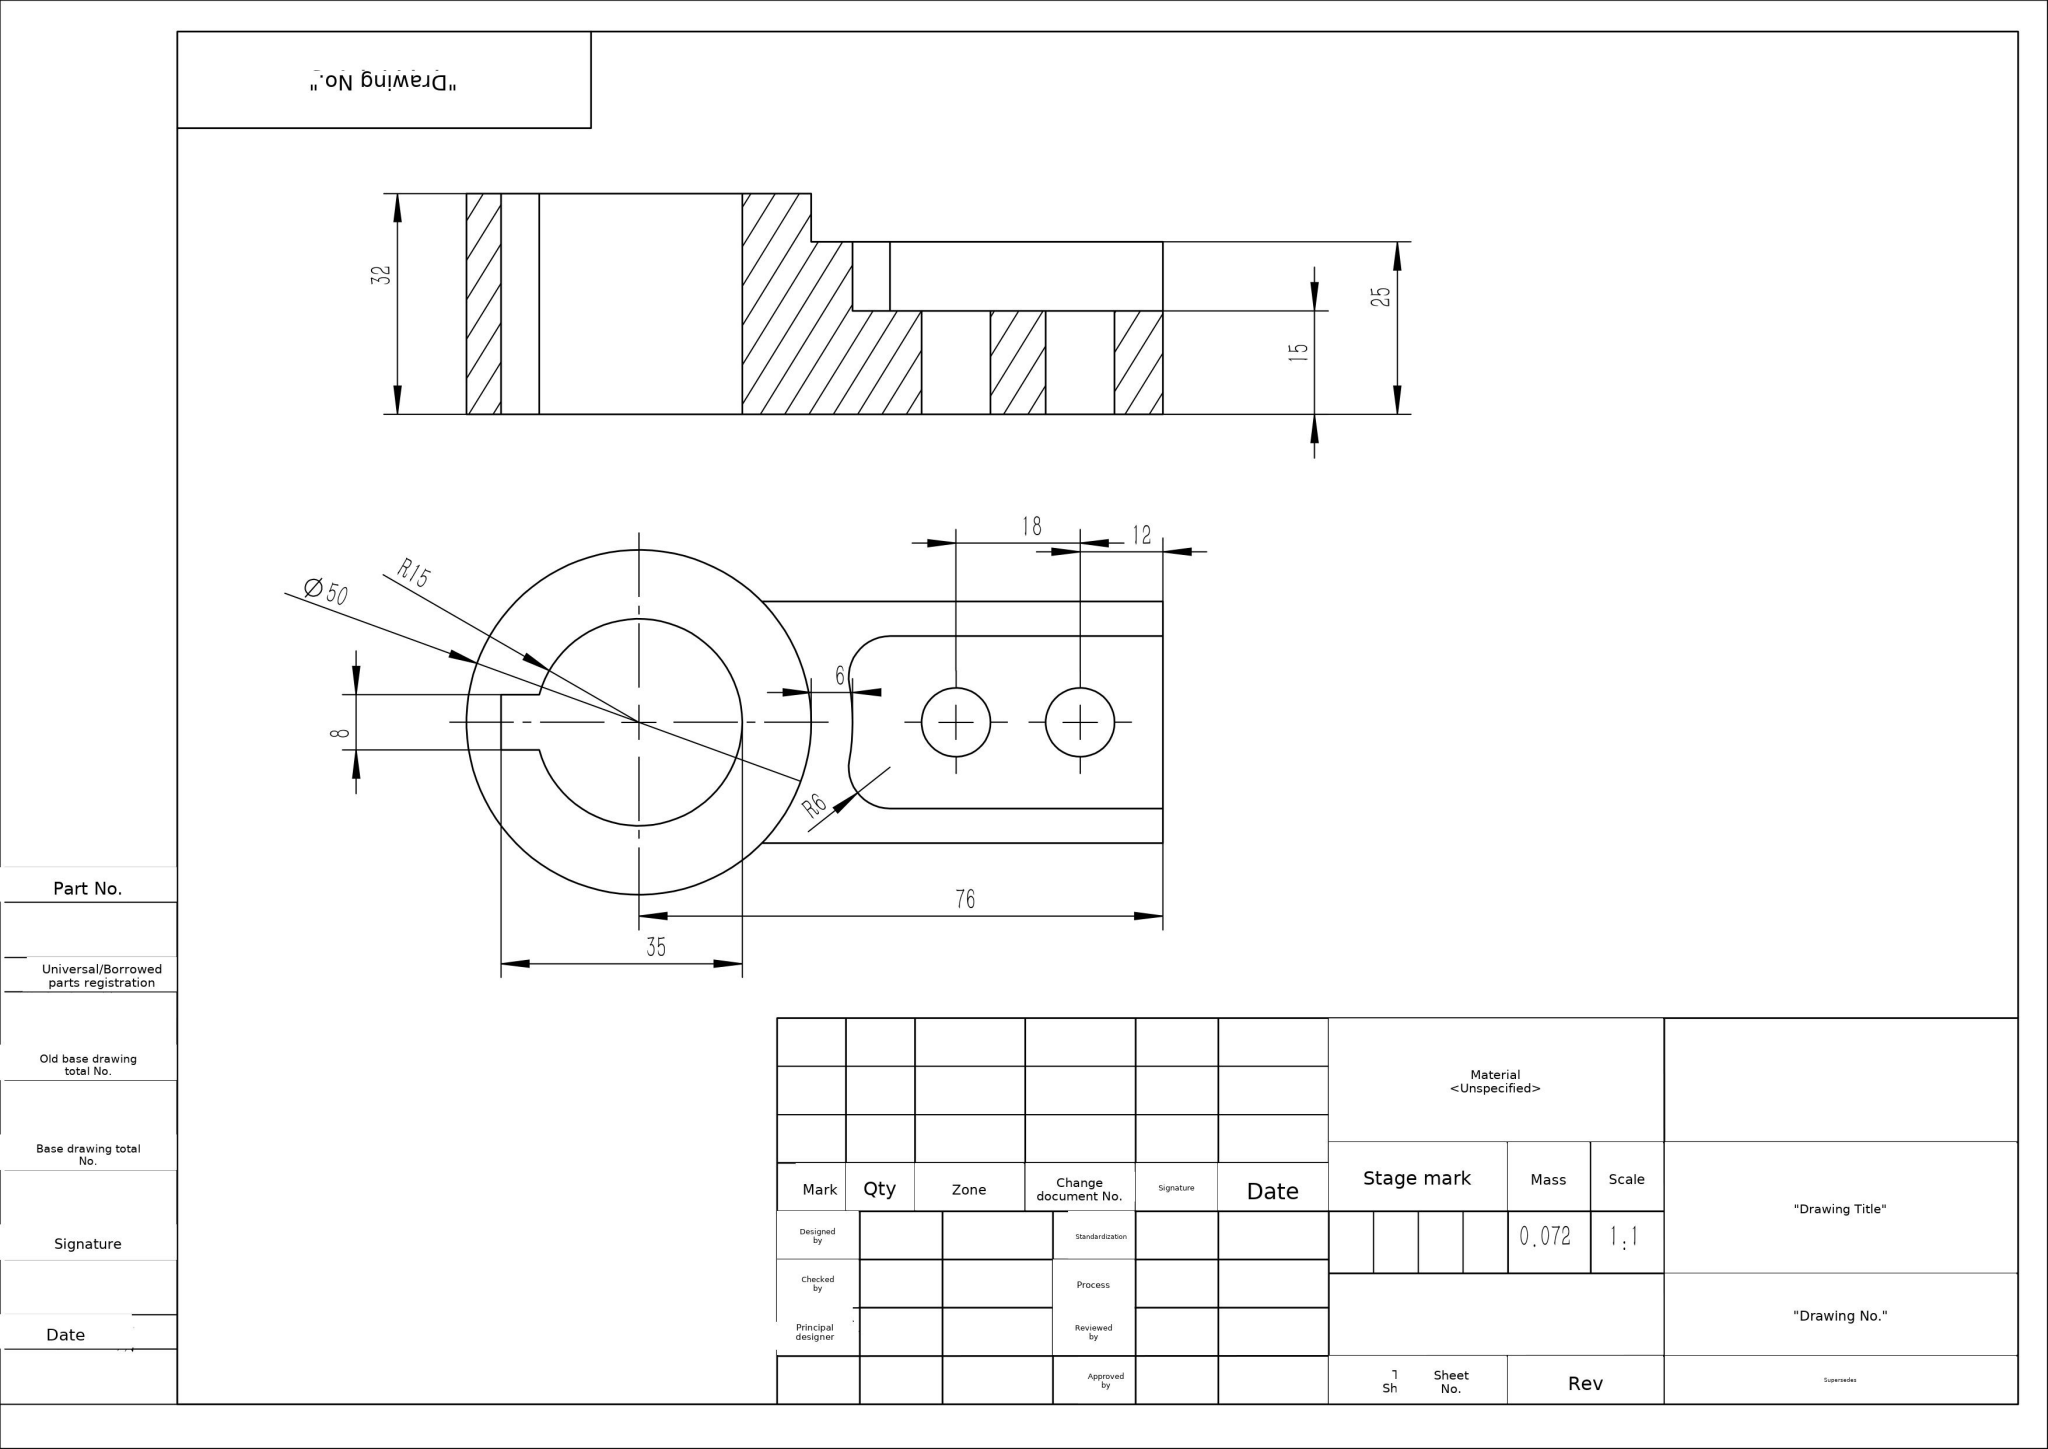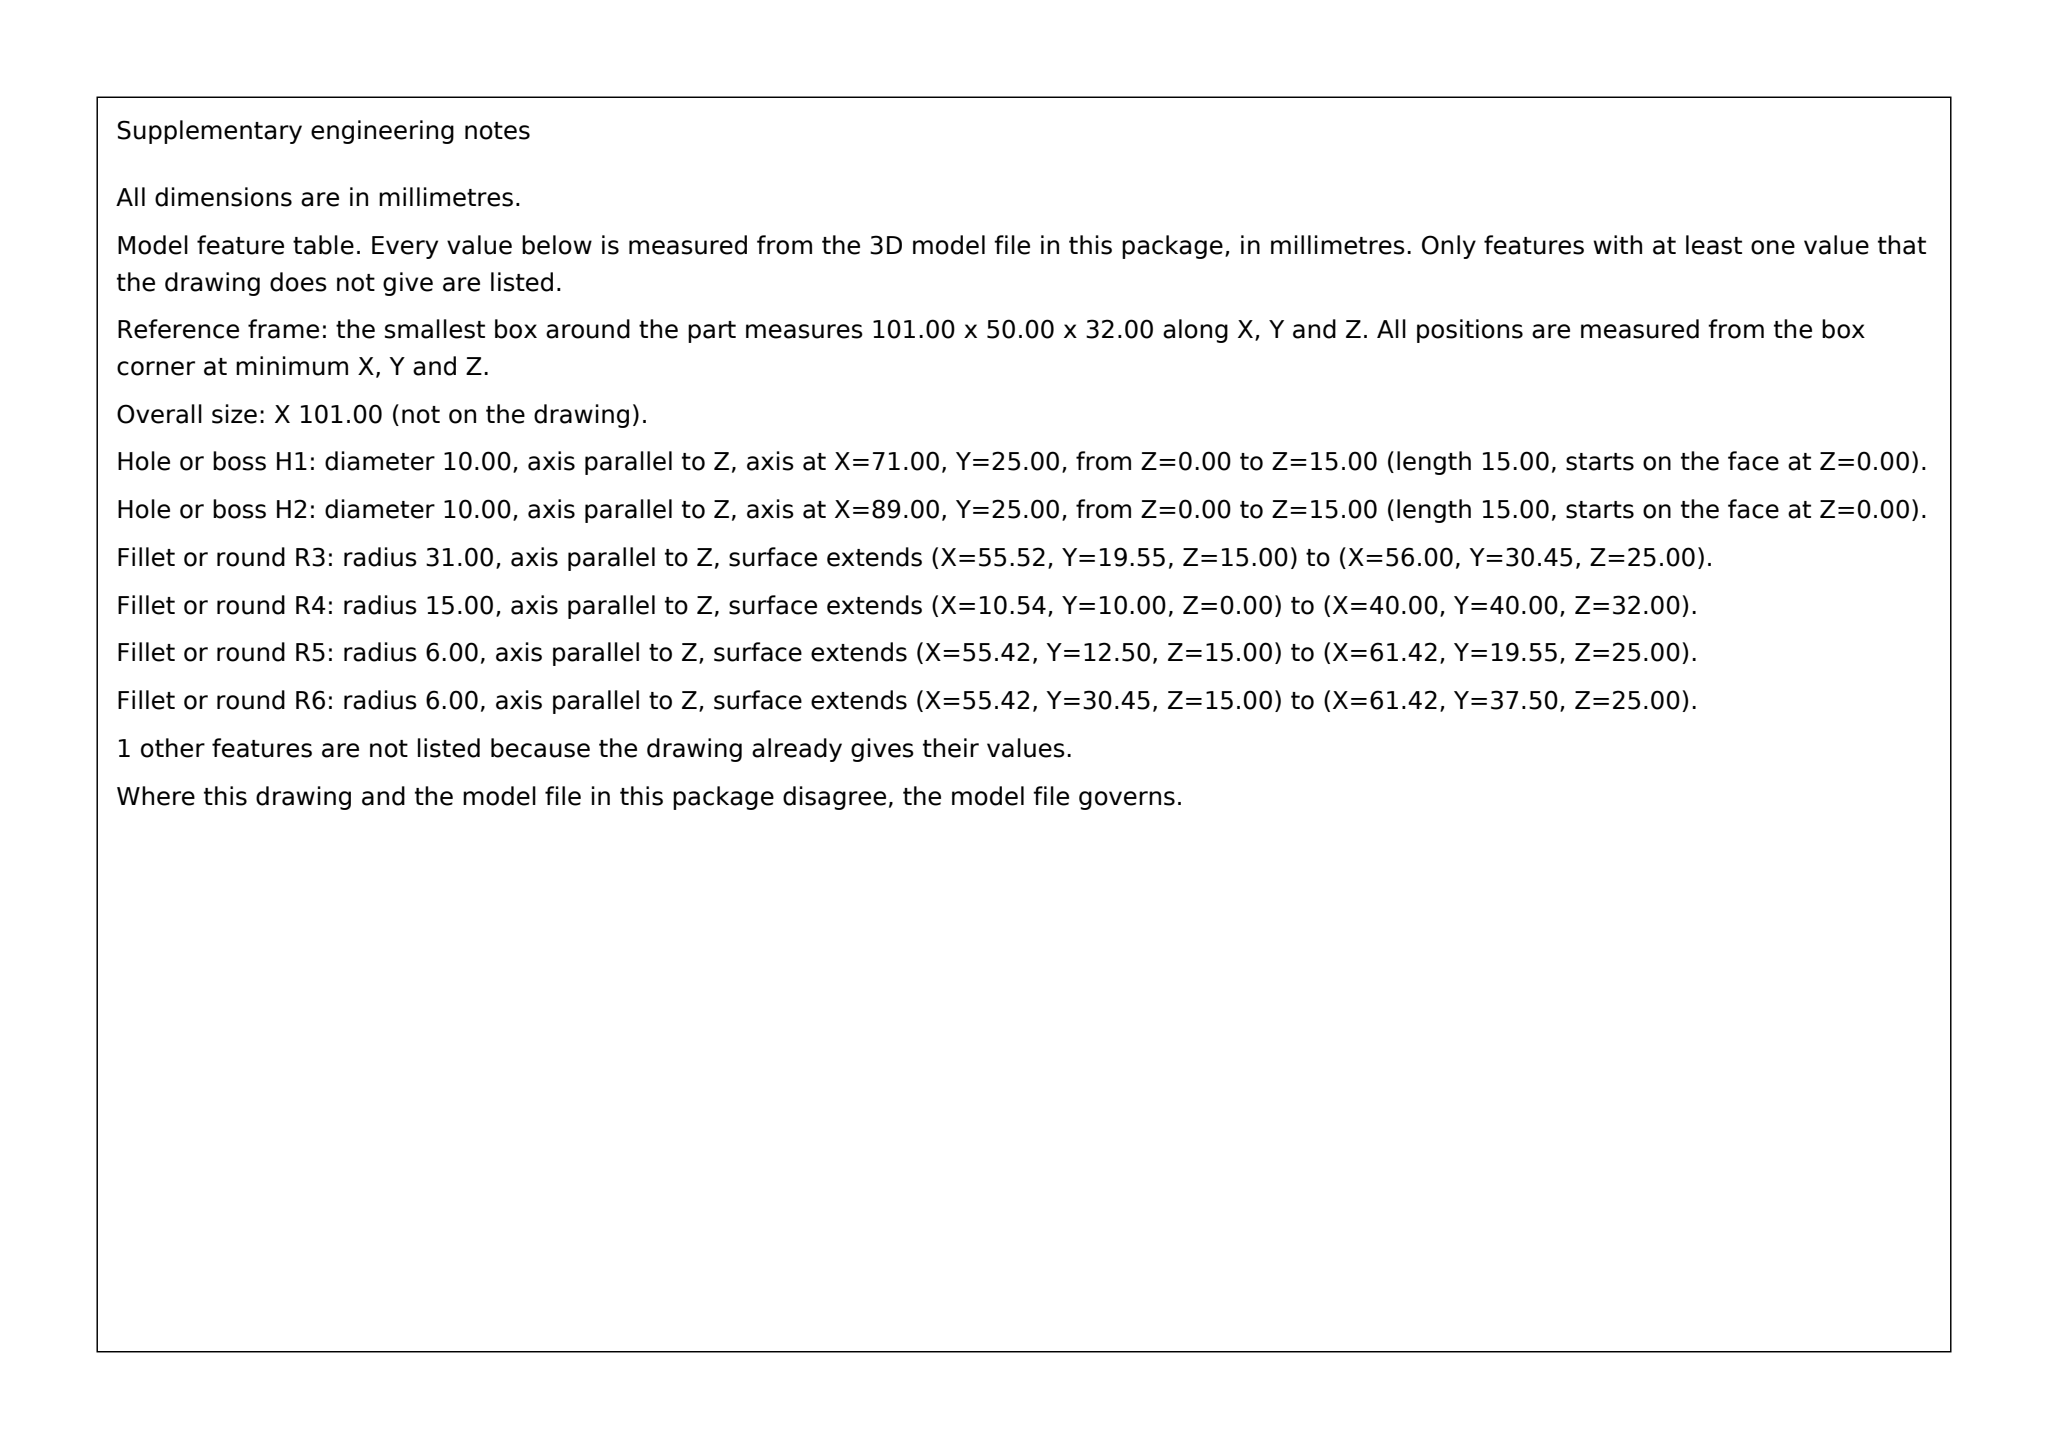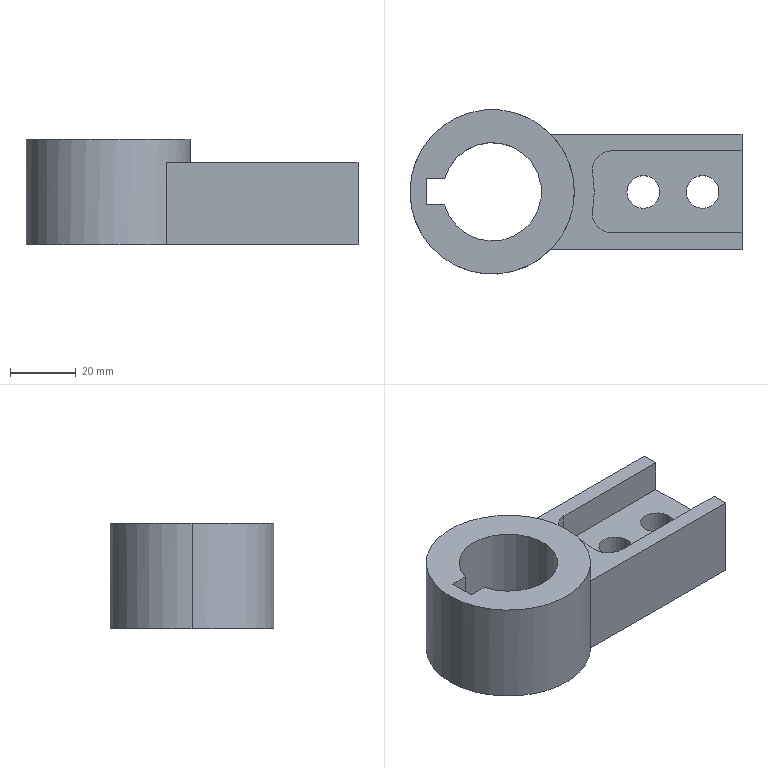Part | SolidWorks | mm | 1 solid | 23 faces | box 101 x 50 x 32 mm | volume 71910 mm3 | plane 12 | cylinder 11 | commonest cylinder face diameters 10 x4 62 x2 50 x2 12 x2 30 x1
build123d program:
from build123d import *

# Parameters (mm, degrees)
SKETCH1_R           = 25
BOSS_EXTRUDE1_DEPTH = 32
SKETCH2_W           = 61
SKETCH2_H           = 35
BOSS_EXTRUDE2_DEPTH = 25
CUT_EXTRUDE1_DEPTH  = 10
SKETCH4_R           = 5
CUT_EXTRUDE2_DEPTH  = 28


with BuildPart() as part:
    # Sketch1 → Boss-Extrude1 (new body)
    with BuildSketch(Plane.XY):
        Circle(SKETCH1_R)
        with BuildLine():
            Line((-14.457, 4), (-20, 4))
            Line((-20, 4), (-20, -4))
            Line((-20, -4), (-14.457, -4))
            ThreePointArc((-14.457, -4), (15, 0), (-14.457, 4))
        make_face(mode=Mode.SUBTRACT)
    extrude(amount=BOSS_EXTRUDE1_DEPTH)

    # Sketch2 → Boss-Extrude2 (add)
    with BuildSketch(Plane(origin=(0, 0, 0), x_dir=(-1, 0, 0), z_dir=(0, 0, -1))):
        with Locations((-45.5, 0)):
            Rectangle(SKETCH2_W, SKETCH2_H)
    extrude(amount=-BOSS_EXTRUDE2_DEPTH)

    # Sketch3 → Cut-Extrude1 (cut)
    with BuildSketch(Plane.XY.offset(25)):
        with BuildLine():
            Line((76, -12.5), (76, 12.5))
            Line((76, 12.5), (36.425, 12.5))
            ThreePointArc((36.425, 12.5), (31.824, 10.352), (30.518, 5.446))
            ThreePointArc((30.518, 5.446), (31, 0), (30.518, -5.446))
            ThreePointArc((30.518, -5.446), (31.824, -10.352), (36.425, -12.5))
            Line((36.425, -12.5), (76, -12.5))
        make_face()
    extrude(amount=-CUT_EXTRUDE1_DEPTH, mode=Mode.SUBTRACT)

    # Sketch4 → Cut-Extrude2 (cut)
    with BuildSketch(Plane.XY.offset(15)):
        with Locations((46, 0)):
            Circle(SKETCH4_R)
        with Locations((64, 0)):
            Circle(SKETCH4_R)
    extrude(amount=-CUT_EXTRUDE2_DEPTH, mode=Mode.SUBTRACT)


solid = part.part
STEP:
#1=CARTESIAN_POINT('',(59.,0.,0.));
#2=VERTEX_POINT('',#1);
#3=CARTESIAN_POINT('',(69.,0.,0.));
#4=VERTEX_POINT('',#3);
#5=CARTESIAN_POINT('',(64.,0.,0.));
#6=DIRECTION('',(0.,0.,1.));
#7=DIRECTION('',(1.,0.,0.));
#8=AXIS2_PLACEMENT_3D('',#5,#6,#7);
#9=CIRCLE('',#8,5.);
#10=EDGE_CURVE('',#2,#4,#9,.T.);
#11=ORIENTED_EDGE('',*,*,#10,.F.);
#12=CARTESIAN_POINT('',(59.,0.,15.));
#13=VERTEX_POINT('',#12);
#14=CARTESIAN_POINT('',(59.,0.,-13.));
#15=DIRECTION('',(0.,0.,1.));
#16=VECTOR('',#15,1000.);
#17=LINE('',#14,#16);
#18=EDGE_CURVE('',#2,#13,#17,.T.);
#19=ORIENTED_EDGE('',*,*,#18,.T.);
#20=CARTESIAN_POINT('',(69.,0.,15.));
#21=VERTEX_POINT('',#20);
#22=CARTESIAN_POINT('',(64.,0.,15.));
#23=DIRECTION('',(0.,0.,1.));
#24=DIRECTION('',(1.,0.,0.));
#25=AXIS2_PLACEMENT_3D('',#22,#23,#24);
#26=CIRCLE('',#25,5.);
#27=EDGE_CURVE('',#13,#21,#26,.T.);
#28=ORIENTED_EDGE('',*,*,#27,.T.);
#29=CARTESIAN_POINT('',(69.,0.,-13.));
#30=DIRECTION('',(0.,0.,1.));
#31=VECTOR('',#30,1000.);
#32=LINE('',#29,#31);
#33=EDGE_CURVE('',#4,#21,#32,.T.);
#34=ORIENTED_EDGE('',*,*,#33,.F.);
#35=EDGE_LOOP('',(#11,#19,#28,#34));
#36=FACE_OUTER_BOUND('',#35,.T.);
#37=CARTESIAN_POINT('',(64.,0.,-13.));
#38=DIRECTION('',(0.,0.,1.));
#39=DIRECTION('',(1.,0.,0.));
#40=AXIS2_PLACEMENT_3D('',#37,#38,#39);
#41=CYLINDRICAL_SURFACE('',#40,5.);
#42=ADVANCED_FACE('',(#36),#41,.F.);
#43=CARTESIAN_POINT('',(41.,0.,0.));
#44=VERTEX_POINT('',#43);
#45=CARTESIAN_POINT('',(51.,0.,0.));
#46=VERTEX_POINT('',#45);
#47=CARTESIAN_POINT('',(46.,0.,0.));
#48=DIRECTION('',(0.,0.,1.));
#49=DIRECTION('',(1.,0.,0.));
#50=AXIS2_PLACEMENT_3D('',#47,#48,#49);
#51=CIRCLE('',#50,5.);
#52=EDGE_CURVE('',#44,#46,#51,.T.);
#53=ORIENTED_EDGE('',*,*,#52,.F.);
#54=CARTESIAN_POINT('',(41.,0.,15.));
#55=VERTEX_POINT('',#54);
#56=CARTESIAN_POINT('',(41.,0.,-13.));
#57=DIRECTION('',(0.,0.,1.));
#58=VECTOR('',#57,1000.);
#59=LINE('',#56,#58);
#60=EDGE_CURVE('',#44,#55,#59,.T.);
#61=ORIENTED_EDGE('',*,*,#60,.T.);
#62=CARTESIAN_POINT('',(51.,0.,15.));
#63=VERTEX_POINT('',#62);
#64=CARTESIAN_POINT('',(46.,0.,15.));
#65=DIRECTION('',(0.,0.,1.));
#66=DIRECTION('',(1.,0.,0.));
#67=AXIS2_PLACEMENT_3D('',#64,#65,#66);
#68=CIRCLE('',#67,5.);
#69=EDGE_CURVE('',#55,#63,#68,.T.);
#70=ORIENTED_EDGE('',*,*,#69,.T.);
#71=CARTESIAN_POINT('',(51.,0.,-13.));
#72=DIRECTION('',(0.,0.,1.));
#73=VECTOR('',#72,1000.);
#74=LINE('',#71,#73);
#75=EDGE_CURVE('',#46,#63,#74,.T.);
#76=ORIENTED_EDGE('',*,*,#75,.F.);
#77=EDGE_LOOP('',(#53,#61,#70,#76));
#78=FACE_OUTER_BOUND('',#77,.T.);
#79=CARTESIAN_POINT('',(46.,0.,-13.));
#80=DIRECTION('',(0.,0.,1.));
#81=DIRECTION('',(1.,0.,0.));
#82=AXIS2_PLACEMENT_3D('',#79,#80,#81);
#83=CYLINDRICAL_SURFACE('',#82,5.);
#84=ADVANCED_FACE('',(#78),#83,.F.);
#85=CARTESIAN_POINT('',(30.518,-5.446,15.));
#86=VERTEX_POINT('',#85);
#87=CARTESIAN_POINT('',(31.,0.,15.));
#88=VERTEX_POINT('',#87);
#89=CARTESIAN_POINT('',(0.,0.,15.));
#90=DIRECTION('',(0.,0.,1.));
#91=DIRECTION('',(1.,0.,0.));
#92=AXIS2_PLACEMENT_3D('',#89,#90,#91);
#93=CIRCLE('',#92,31.);
#94=EDGE_CURVE('',#86,#88,#93,.T.);
#95=ORIENTED_EDGE('',*,*,#94,.T.);
#96=CARTESIAN_POINT('',(31.,0.,25.));
#97=VERTEX_POINT('',#96);
#98=CARTESIAN_POINT('',(31.,0.,15.));
#99=DIRECTION('',(0.,0.,1.));
#100=VECTOR('',#99,1000.);
#101=LINE('',#98,#100);
#102=EDGE_CURVE('',#88,#97,#101,.T.);
#103=ORIENTED_EDGE('',*,*,#102,.T.);
#104=CARTESIAN_POINT('',(30.518,-5.446,25.));
#105=VERTEX_POINT('',#104);
#106=CARTESIAN_POINT('',(0.,0.,25.));
#107=DIRECTION('',(0.,0.,1.));
#108=DIRECTION('',(1.,0.,0.));
#109=AXIS2_PLACEMENT_3D('',#106,#107,#108);
#110=CIRCLE('',#109,31.);
#111=EDGE_CURVE('',#105,#97,#110,.T.);
#112=ORIENTED_EDGE('',*,*,#111,.F.);
#113=CARTESIAN_POINT('',(30.518,-5.446,15.));
#114=DIRECTION('',(0.,0.,1.));
#115=VECTOR('',#114,1000.);
#116=LINE('',#113,#115);
#117=EDGE_CURVE('',#86,#105,#116,.T.);
#118=ORIENTED_EDGE('',*,*,#117,.F.);
#119=EDGE_LOOP('',(#95,#103,#112,#118));
#120=FACE_OUTER_BOUND('',#119,.T.);
#121=CARTESIAN_POINT('',(0.,0.,15.));
#122=DIRECTION('',(0.,0.,1.));
#123=DIRECTION('',(1.,0.,0.));
#124=AXIS2_PLACEMENT_3D('',#121,#122,#123);
#125=CYLINDRICAL_SURFACE('',#124,31.);
#126=ADVANCED_FACE('',(#120),#125,.T.);
#127=CARTESIAN_POINT('',(25.,0.,32.));
#128=VERTEX_POINT('',#127);
#129=CARTESIAN_POINT('',(-25.,0.,32.));
#130=VERTEX_POINT('',#129);
#131=CARTESIAN_POINT('',(0.,0.,32.));
#132=DIRECTION('',(0.,0.,1.));
#133=DIRECTION('',(1.,0.,0.));
#134=AXIS2_PLACEMENT_3D('',#131,#132,#133);
#135=CIRCLE('',#134,25.);
#136=EDGE_CURVE('',#128,#130,#135,.T.);
#137=ORIENTED_EDGE('',*,*,#136,.F.);
#138=CARTESIAN_POINT('',(25.,0.,25.));
#139=VERTEX_POINT('',#138);
#140=CARTESIAN_POINT('',(25.,0.,32.));
#141=DIRECTION('',(0.,0.,-1.));
#142=VECTOR('',#141,1000.);
#143=LINE('',#140,#142);
#144=EDGE_CURVE('',#128,#139,#143,.T.);
#145=ORIENTED_EDGE('',*,*,#144,.T.);
#146=CARTESIAN_POINT('',(17.854,17.5,25.));
#147=VERTEX_POINT('',#146);
#148=CARTESIAN_POINT('',(0.,0.,25.));
#149=DIRECTION('',(0.,0.,1.));
#150=DIRECTION('',(1.,0.,0.));
#151=AXIS2_PLACEMENT_3D('',#148,#149,#150);
#152=CIRCLE('',#151,25.);
#153=EDGE_CURVE('',#139,#147,#152,.T.);
#154=ORIENTED_EDGE('',*,*,#153,.T.);
#155=CARTESIAN_POINT('',(17.854,17.5,0.));
#156=VERTEX_POINT('',#155);
#157=CARTESIAN_POINT('',(17.854,17.5,32.));
#158=DIRECTION('',(0.,0.,-1.));
#159=VECTOR('',#158,1000.);
#160=LINE('',#157,#159);
#161=EDGE_CURVE('',#147,#156,#160,.T.);
#162=ORIENTED_EDGE('',*,*,#161,.T.);
#163=CARTESIAN_POINT('',(-25.,0.,0.));
#164=VERTEX_POINT('',#163);
#165=CARTESIAN_POINT('',(0.,0.,0.));
#166=DIRECTION('',(0.,0.,1.));
#167=DIRECTION('',(1.,0.,0.));
#168=AXIS2_PLACEMENT_3D('',#165,#166,#167);
#169=CIRCLE('',#168,25.);
#170=EDGE_CURVE('',#156,#164,#169,.T.);
#171=ORIENTED_EDGE('',*,*,#170,.T.);
#172=CARTESIAN_POINT('',(-25.,0.,32.));
#173=DIRECTION('',(0.,0.,-1.));
#174=VECTOR('',#173,1000.);
#175=LINE('',#172,#174);
#176=EDGE_CURVE('',#130,#164,#175,.T.);
#177=ORIENTED_EDGE('',*,*,#176,.F.);
#178=EDGE_LOOP('',(#137,#145,#154,#162,#171,#177));
#179=FACE_OUTER_BOUND('',#178,.T.);
#180=CARTESIAN_POINT('',(0.,0.,32.));
#181=DIRECTION('',(0.,0.,-1.));
#182=DIRECTION('',(-1.,0.,0.));
#183=AXIS2_PLACEMENT_3D('',#180,#181,#182);
#184=CYLINDRICAL_SURFACE('',#183,25.);
#185=ADVANCED_FACE('',(#179),#184,.T.);
#186=CARTESIAN_POINT('',(0.,0.,32.));
#187=DIRECTION('',(0.,0.,1.));
#188=DIRECTION('',(1.,0.,0.));
#189=AXIS2_PLACEMENT_3D('',#186,#187,#188);
#190=CIRCLE('',#189,25.);
#191=EDGE_CURVE('',#130,#128,#190,.T.);
#192=ORIENTED_EDGE('',*,*,#191,.T.);
#193=ORIENTED_EDGE('',*,*,#136,.T.);
#194=EDGE_LOOP('',(#192,#193));
#195=FACE_OUTER_BOUND('',#194,.T.);
#196=CARTESIAN_POINT('',(-20.,-4.,32.));
#197=VERTEX_POINT('',#196);
#198=CARTESIAN_POINT('',(-14.457,-4.,32.));
#199=VERTEX_POINT('',#198);
#200=CARTESIAN_POINT('',(-14.457,-4.,32.));
#201=DIRECTION('',(1.,0.,0.));
#202=VECTOR('',#201,1000.);
#203=LINE('',#200,#202);
#204=EDGE_CURVE('',#197,#199,#203,.T.);
#205=ORIENTED_EDGE('',*,*,#204,.F.);
#206=CARTESIAN_POINT('',(-20.,4.,32.));
#207=VERTEX_POINT('',#206);
#208=CARTESIAN_POINT('',(-20.,4.,32.));
#209=DIRECTION('',(0.,-1.,0.));
#210=VECTOR('',#209,1000.);
#211=LINE('',#208,#210);
#212=EDGE_CURVE('',#207,#197,#211,.T.);
#213=ORIENTED_EDGE('',*,*,#212,.F.);
#214=CARTESIAN_POINT('',(-14.457,4.,32.));
#215=VERTEX_POINT('',#214);
#216=CARTESIAN_POINT('',(-14.457,4.,32.));
#217=DIRECTION('',(-1.,-0.,0.));
#218=VECTOR('',#217,1000.);
#219=LINE('',#216,#218);
#220=EDGE_CURVE('',#215,#207,#219,.T.);
#221=ORIENTED_EDGE('',*,*,#220,.F.);
#222=CARTESIAN_POINT('',(0.,0.,32.));
#223=DIRECTION('',(0.,0.,1.));
#224=DIRECTION('',(1.,0.,0.));
#225=AXIS2_PLACEMENT_3D('',#222,#223,#224);
#226=CIRCLE('',#225,15.);
#227=EDGE_CURVE('',#199,#215,#226,.T.);
#228=ORIENTED_EDGE('',*,*,#227,.F.);
#229=EDGE_LOOP('',(#205,#213,#221,#228));
#230=FACE_BOUND('',#229,.T.);
#231=CARTESIAN_POINT('',(0.,0.,32.));
#232=DIRECTION('',(0.,0.,1.));
#233=DIRECTION('',(1.,0.,0.));
#234=AXIS2_PLACEMENT_3D('',#231,#232,#233);
#235=PLANE('',#234);
#236=ADVANCED_FACE('',(#195,#230),#235,.T.);
#237=CARTESIAN_POINT('',(64.,0.,0.));
#238=DIRECTION('',(0.,0.,1.));
#239=DIRECTION('',(1.,0.,0.));
#240=AXIS2_PLACEMENT_3D('',#237,#238,#239);
#241=CIRCLE('',#240,5.);
#242=EDGE_CURVE('',#4,#2,#241,.T.);
#243=ORIENTED_EDGE('',*,*,#242,.T.);
#244=ORIENTED_EDGE('',*,*,#10,.T.);
#245=EDGE_LOOP('',(#243,#244));
#246=FACE_BOUND('',#245,.T.);
#247=CARTESIAN_POINT('',(46.,0.,0.));
#248=DIRECTION('',(0.,0.,1.));
#249=DIRECTION('',(1.,0.,0.));
#250=AXIS2_PLACEMENT_3D('',#247,#248,#249);
#251=CIRCLE('',#250,5.);
#252=EDGE_CURVE('',#46,#44,#251,.T.);
#253=ORIENTED_EDGE('',*,*,#252,.T.);
#254=ORIENTED_EDGE('',*,*,#52,.T.);
#255=EDGE_LOOP('',(#253,#254));
#256=FACE_BOUND('',#255,.T.);
#257=CARTESIAN_POINT('',(-14.457,-4.,0.));
#258=VERTEX_POINT('',#257);
#259=CARTESIAN_POINT('',(-14.457,4.,0.));
#260=VERTEX_POINT('',#259);
#261=CARTESIAN_POINT('',(0.,0.,0.));
#262=DIRECTION('',(0.,0.,1.));
#263=DIRECTION('',(1.,0.,0.));
#264=AXIS2_PLACEMENT_3D('',#261,#262,#263);
#265=CIRCLE('',#264,15.);
#266=EDGE_CURVE('',#258,#260,#265,.T.);
#267=ORIENTED_EDGE('',*,*,#266,.T.);
#268=CARTESIAN_POINT('',(-20.,4.,0.));
#269=VERTEX_POINT('',#268);
#270=CARTESIAN_POINT('',(-14.457,4.,0.));
#271=DIRECTION('',(-1.,-0.,0.));
#272=VECTOR('',#271,1000.);
#273=LINE('',#270,#272);
#274=EDGE_CURVE('',#260,#269,#273,.T.);
#275=ORIENTED_EDGE('',*,*,#274,.T.);
#276=CARTESIAN_POINT('',(-20.,-4.,0.));
#277=VERTEX_POINT('',#276);
#278=CARTESIAN_POINT('',(-20.,4.,0.));
#279=DIRECTION('',(0.,-1.,0.));
#280=VECTOR('',#279,1000.);
#281=LINE('',#278,#280);
#282=EDGE_CURVE('',#269,#277,#281,.T.);
#283=ORIENTED_EDGE('',*,*,#282,.T.);
#284=CARTESIAN_POINT('',(-14.457,-4.,0.));
#285=DIRECTION('',(1.,0.,0.));
#286=VECTOR('',#285,1000.);
#287=LINE('',#284,#286);
#288=EDGE_CURVE('',#277,#258,#287,.T.);
#289=ORIENTED_EDGE('',*,*,#288,.T.);
#290=EDGE_LOOP('',(#267,#275,#283,#289));
#291=FACE_BOUND('',#290,.T.);
#292=CARTESIAN_POINT('',(76.,-17.5,0.));
#293=VERTEX_POINT('',#292);
#294=CARTESIAN_POINT('',(17.854,-17.5,0.));
#295=VERTEX_POINT('',#294);
#296=CARTESIAN_POINT('',(15.,-17.5,0.));
#297=DIRECTION('',(-1.,0.,0.));
#298=VECTOR('',#297,1000.);
#299=LINE('',#296,#298);
#300=EDGE_CURVE('',#293,#295,#299,.T.);
#301=ORIENTED_EDGE('',*,*,#300,.T.);
#302=CARTESIAN_POINT('',(0.,0.,0.));
#303=DIRECTION('',(0.,0.,1.));
#304=DIRECTION('',(1.,0.,0.));
#305=AXIS2_PLACEMENT_3D('',#302,#303,#304);
#306=CIRCLE('',#305,25.);
#307=EDGE_CURVE('',#164,#295,#306,.T.);
#308=ORIENTED_EDGE('',*,*,#307,.F.);
#309=ORIENTED_EDGE('',*,*,#170,.F.);
#310=CARTESIAN_POINT('',(76.,17.5,0.));
#311=VERTEX_POINT('',#310);
#312=CARTESIAN_POINT('',(15.,17.5,0.));
#313=DIRECTION('',(1.,0.,0.));
#314=VECTOR('',#313,1000.);
#315=LINE('',#312,#314);
#316=EDGE_CURVE('',#156,#311,#315,.T.);
#317=ORIENTED_EDGE('',*,*,#316,.T.);
#318=CARTESIAN_POINT('',(76.,17.5,0.));
#319=DIRECTION('',(0.,-1.,0.));
#320=VECTOR('',#319,1000.);
#321=LINE('',#318,#320);
#322=EDGE_CURVE('',#311,#293,#321,.T.);
#323=ORIENTED_EDGE('',*,*,#322,.T.);
#324=EDGE_LOOP('',(#301,#308,#309,#317,#323));
#325=FACE_OUTER_BOUND('',#324,.T.);
#326=CARTESIAN_POINT('',(0.,0.,0.));
#327=DIRECTION('',(0.,0.,1.));
#328=DIRECTION('',(1.,0.,0.));
#329=AXIS2_PLACEMENT_3D('',#326,#327,#328);
#330=PLANE('',#329);
#331=ADVANCED_FACE('',(#246,#256,#291,#325),#330,.F.);
#332=ORIENTED_EDGE('',*,*,#144,.F.);
#333=ORIENTED_EDGE('',*,*,#191,.F.);
#334=ORIENTED_EDGE('',*,*,#176,.T.);
#335=ORIENTED_EDGE('',*,*,#307,.T.);
#336=CARTESIAN_POINT('',(17.854,-17.5,25.));
#337=VERTEX_POINT('',#336);
#338=CARTESIAN_POINT('',(17.854,-17.5,32.));
#339=DIRECTION('',(0.,0.,1.));
#340=VECTOR('',#339,1000.);
#341=LINE('',#338,#340);
#342=EDGE_CURVE('',#295,#337,#341,.T.);
#343=ORIENTED_EDGE('',*,*,#342,.T.);
#344=CARTESIAN_POINT('',(0.,0.,25.));
#345=DIRECTION('',(0.,0.,1.));
#346=DIRECTION('',(1.,0.,0.));
#347=AXIS2_PLACEMENT_3D('',#344,#345,#346);
#348=CIRCLE('',#347,25.);
#349=EDGE_CURVE('',#337,#139,#348,.T.);
#350=ORIENTED_EDGE('',*,*,#349,.T.);
#351=EDGE_LOOP('',(#332,#333,#334,#335,#343,#350));
#352=FACE_OUTER_BOUND('',#351,.T.);
#353=CARTESIAN_POINT('',(0.,0.,32.));
#354=DIRECTION('',(0.,0.,-1.));
#355=DIRECTION('',(-1.,0.,0.));
#356=AXIS2_PLACEMENT_3D('',#353,#354,#355);
#357=CYLINDRICAL_SURFACE('',#356,25.);
#358=ADVANCED_FACE('',(#352),#357,.T.);
#359=ORIENTED_EDGE('',*,*,#282,.F.);
#360=CARTESIAN_POINT('',(-20.,4.,32.));
#361=DIRECTION('',(0.,0.,-1.));
#362=VECTOR('',#361,1000.);
#363=LINE('',#360,#362);
#364=EDGE_CURVE('',#207,#269,#363,.T.);
#365=ORIENTED_EDGE('',*,*,#364,.F.);
#366=ORIENTED_EDGE('',*,*,#212,.T.);
#367=CARTESIAN_POINT('',(-20.,-4.,32.));
#368=DIRECTION('',(0.,0.,-1.));
#369=VECTOR('',#368,1000.);
#370=LINE('',#367,#369);
#371=EDGE_CURVE('',#197,#277,#370,.T.);
#372=ORIENTED_EDGE('',*,*,#371,.T.);
#373=EDGE_LOOP('',(#359,#365,#366,#372));
#374=FACE_OUTER_BOUND('',#373,.T.);
#375=CARTESIAN_POINT('',(-20.,4.,32.));
#376=DIRECTION('',(1.,0.,0.));
#377=DIRECTION('',(-0.,1.,0.));
#378=AXIS2_PLACEMENT_3D('',#375,#376,#377);
#379=PLANE('',#378);
#380=ADVANCED_FACE('',(#374),#379,.T.);
#381=ORIENTED_EDGE('',*,*,#288,.F.);
#382=ORIENTED_EDGE('',*,*,#371,.F.);
#383=ORIENTED_EDGE('',*,*,#204,.T.);
#384=CARTESIAN_POINT('',(-14.457,-4.,32.));
#385=DIRECTION('',(0.,0.,-1.));
#386=VECTOR('',#385,1000.);
#387=LINE('',#384,#386);
#388=EDGE_CURVE('',#199,#258,#387,.T.);
#389=ORIENTED_EDGE('',*,*,#388,.T.);
#390=EDGE_LOOP('',(#381,#382,#383,#389));
#391=FACE_OUTER_BOUND('',#390,.T.);
#392=CARTESIAN_POINT('',(-14.457,-4.,32.));
#393=DIRECTION('',(-0.,1.,0.));
#394=DIRECTION('',(-1.,-0.,0.));
#395=AXIS2_PLACEMENT_3D('',#392,#393,#394);
#396=PLANE('',#395);
#397=ADVANCED_FACE('',(#391),#396,.T.);
#398=CARTESIAN_POINT('',(-14.457,4.,32.));
#399=DIRECTION('',(0.,0.,-1.));
#400=VECTOR('',#399,1000.);
#401=LINE('',#398,#400);
#402=EDGE_CURVE('',#215,#260,#401,.T.);
#403=ORIENTED_EDGE('',*,*,#402,.T.);
#404=ORIENTED_EDGE('',*,*,#266,.F.);
#405=ORIENTED_EDGE('',*,*,#388,.F.);
#406=ORIENTED_EDGE('',*,*,#227,.T.);
#407=EDGE_LOOP('',(#403,#404,#405,#406));
#408=FACE_OUTER_BOUND('',#407,.T.);
#409=CARTESIAN_POINT('',(0.,0.,32.));
#410=DIRECTION('',(0.,0.,-1.));
#411=DIRECTION('',(-1.,0.,0.));
#412=AXIS2_PLACEMENT_3D('',#409,#410,#411);
#413=CYLINDRICAL_SURFACE('',#412,15.);
#414=ADVANCED_FACE('',(#408),#413,.F.);
#415=ORIENTED_EDGE('',*,*,#274,.F.);
#416=ORIENTED_EDGE('',*,*,#402,.F.);
#417=ORIENTED_EDGE('',*,*,#220,.T.);
#418=ORIENTED_EDGE('',*,*,#364,.T.);
#419=EDGE_LOOP('',(#415,#416,#417,#418));
#420=FACE_OUTER_BOUND('',#419,.T.);
#421=CARTESIAN_POINT('',(-14.457,4.,32.));
#422=DIRECTION('',(0.,-1.,0.));
#423=DIRECTION('',(1.,0.,0.));
#424=AXIS2_PLACEMENT_3D('',#421,#422,#423);
#425=PLANE('',#424);
#426=ADVANCED_FACE('',(#420),#425,.T.);
#427=ORIENTED_EDGE('',*,*,#342,.F.);
#428=ORIENTED_EDGE('',*,*,#300,.F.);
#429=CARTESIAN_POINT('',(76.,-17.5,25.));
#430=VERTEX_POINT('',#429);
#431=CARTESIAN_POINT('',(76.,-17.5,25.));
#432=DIRECTION('',(0.,0.,-1.));
#433=VECTOR('',#432,1000.);
#434=LINE('',#431,#433);
#435=EDGE_CURVE('',#430,#293,#434,.T.);
#436=ORIENTED_EDGE('',*,*,#435,.F.);
#437=CARTESIAN_POINT('',(15.,-17.5,25.));
#438=DIRECTION('',(-1.,0.,0.));
#439=VECTOR('',#438,1000.);
#440=LINE('',#437,#439);
#441=EDGE_CURVE('',#430,#337,#440,.T.);
#442=ORIENTED_EDGE('',*,*,#441,.T.);
#443=EDGE_LOOP('',(#427,#428,#436,#442));
#444=FACE_OUTER_BOUND('',#443,.T.);
#445=CARTESIAN_POINT('',(15.,-17.5,25.));
#446=DIRECTION('',(-0.,-1.,0.));
#447=DIRECTION('',(1.,-0.,0.));
#448=AXIS2_PLACEMENT_3D('',#445,#446,#447);
#449=PLANE('',#448);
#450=ADVANCED_FACE('',(#444),#449,.T.);
#451=ORIENTED_EDGE('',*,*,#161,.F.);
#452=CARTESIAN_POINT('',(76.,17.5,25.));
#453=VERTEX_POINT('',#452);
#454=CARTESIAN_POINT('',(15.,17.5,25.));
#455=DIRECTION('',(1.,0.,0.));
#456=VECTOR('',#455,1000.);
#457=LINE('',#454,#456);
#458=EDGE_CURVE('',#147,#453,#457,.T.);
#459=ORIENTED_EDGE('',*,*,#458,.T.);
#460=CARTESIAN_POINT('',(76.,17.5,25.));
#461=DIRECTION('',(0.,0.,-1.));
#462=VECTOR('',#461,1000.);
#463=LINE('',#460,#462);
#464=EDGE_CURVE('',#453,#311,#463,.T.);
#465=ORIENTED_EDGE('',*,*,#464,.T.);
#466=ORIENTED_EDGE('',*,*,#316,.F.);
#467=EDGE_LOOP('',(#451,#459,#465,#466));
#468=FACE_OUTER_BOUND('',#467,.T.);
#469=CARTESIAN_POINT('',(15.,17.5,25.));
#470=DIRECTION('',(-0.,1.,0.));
#471=DIRECTION('',(-1.,-0.,0.));
#472=AXIS2_PLACEMENT_3D('',#469,#470,#471);
#473=PLANE('',#472);
#474=ADVANCED_FACE('',(#468),#473,.T.);
#475=CARTESIAN_POINT('',(76.,12.5,25.));
#476=VERTEX_POINT('',#475);
#477=CARTESIAN_POINT('',(36.425,12.5,25.));
#478=VERTEX_POINT('',#477);
#479=CARTESIAN_POINT('',(-0.,12.5,25.));
#480=DIRECTION('',(-1.,-0.,0.));
#481=VECTOR('',#480,1000.);
#482=LINE('',#479,#481);
#483=EDGE_CURVE('',#476,#478,#482,.T.);
#484=ORIENTED_EDGE('',*,*,#483,.F.);
#485=CARTESIAN_POINT('',(76.,17.5,25.));
#486=DIRECTION('',(0.,-1.,0.));
#487=VECTOR('',#486,1000.);
#488=LINE('',#485,#487);
#489=EDGE_CURVE('',#453,#476,#488,.T.);
#490=ORIENTED_EDGE('',*,*,#489,.F.);
#491=ORIENTED_EDGE('',*,*,#458,.F.);
#492=ORIENTED_EDGE('',*,*,#153,.F.);
#493=ORIENTED_EDGE('',*,*,#349,.F.);
#494=ORIENTED_EDGE('',*,*,#441,.F.);
#495=CARTESIAN_POINT('',(76.,-12.5,25.));
#496=VERTEX_POINT('',#495);
#497=CARTESIAN_POINT('',(76.,17.5,25.));
#498=DIRECTION('',(0.,-1.,0.));
#499=VECTOR('',#498,1000.);
#500=LINE('',#497,#499);
#501=EDGE_CURVE('',#496,#430,#500,.T.);
#502=ORIENTED_EDGE('',*,*,#501,.F.);
#503=CARTESIAN_POINT('',(36.425,-12.5,25.));
#504=VERTEX_POINT('',#503);
#505=CARTESIAN_POINT('',(0.,-12.5,25.));
#506=DIRECTION('',(1.,0.,0.));
#507=VECTOR('',#506,1000.);
#508=LINE('',#505,#507);
#509=EDGE_CURVE('',#504,#496,#508,.T.);
#510=ORIENTED_EDGE('',*,*,#509,.F.);
#511=CARTESIAN_POINT('',(36.425,-6.5,25.));
#512=DIRECTION('',(0.,0.,1.));
#513=DIRECTION('',(1.,0.,0.));
#514=AXIS2_PLACEMENT_3D('',#511,#512,#513);
#515=CIRCLE('',#514,6.);
#516=EDGE_CURVE('',#105,#504,#515,.T.);
#517=ORIENTED_EDGE('',*,*,#516,.F.);
#518=ORIENTED_EDGE('',*,*,#111,.T.);
#519=CARTESIAN_POINT('',(30.518,5.446,25.));
#520=VERTEX_POINT('',#519);
#521=CARTESIAN_POINT('',(0.,0.,25.));
#522=DIRECTION('',(0.,0.,1.));
#523=DIRECTION('',(1.,0.,0.));
#524=AXIS2_PLACEMENT_3D('',#521,#522,#523);
#525=CIRCLE('',#524,31.);
#526=EDGE_CURVE('',#97,#520,#525,.T.);
#527=ORIENTED_EDGE('',*,*,#526,.T.);
#528=CARTESIAN_POINT('',(36.425,6.5,25.));
#529=DIRECTION('',(0.,0.,-1.));
#530=DIRECTION('',(1.,0.,0.));
#531=AXIS2_PLACEMENT_3D('',#528,#529,#530);
#532=CIRCLE('',#531,6.);
#533=EDGE_CURVE('',#520,#478,#532,.T.);
#534=ORIENTED_EDGE('',*,*,#533,.T.);
#535=EDGE_LOOP('',(#484,#490,#491,#492,#493,#494,#502,#510,#517,#518,#527,#534));
#536=FACE_OUTER_BOUND('',#535,.T.);
#537=CARTESIAN_POINT('',(0.,0.,25.));
#538=DIRECTION('',(0.,0.,1.));
#539=DIRECTION('',(1.,0.,0.));
#540=AXIS2_PLACEMENT_3D('',#537,#538,#539);
#541=PLANE('',#540);
#542=ADVANCED_FACE('',(#536),#541,.T.);
#543=CARTESIAN_POINT('',(76.,12.5,15.));
#544=VERTEX_POINT('',#543);
#545=CARTESIAN_POINT('',(76.,12.5,15.));
#546=DIRECTION('',(0.,0.,1.));
#547=VECTOR('',#546,1000.);
#548=LINE('',#545,#547);
#549=EDGE_CURVE('',#544,#476,#548,.T.);
#550=ORIENTED_EDGE('',*,*,#549,.F.);
#551=CARTESIAN_POINT('',(76.,-12.5,15.));
#552=VERTEX_POINT('',#551);
#553=CARTESIAN_POINT('',(76.,0.,15.));
#554=DIRECTION('',(0.,1.,0.));
#555=VECTOR('',#554,1000.);
#556=LINE('',#553,#555);
#557=EDGE_CURVE('',#552,#544,#556,.T.);
#558=ORIENTED_EDGE('',*,*,#557,.F.);
#559=CARTESIAN_POINT('',(76.,-12.5,15.));
#560=DIRECTION('',(0.,0.,1.));
#561=VECTOR('',#560,1000.);
#562=LINE('',#559,#561);
#563=EDGE_CURVE('',#552,#496,#562,.T.);
#564=ORIENTED_EDGE('',*,*,#563,.T.);
#565=ORIENTED_EDGE('',*,*,#501,.T.);
#566=ORIENTED_EDGE('',*,*,#435,.T.);
#567=ORIENTED_EDGE('',*,*,#322,.F.);
#568=ORIENTED_EDGE('',*,*,#464,.F.);
#569=ORIENTED_EDGE('',*,*,#489,.T.);
#570=EDGE_LOOP('',(#550,#558,#564,#565,#566,#567,#568,#569));
#571=FACE_OUTER_BOUND('',#570,.T.);
#572=CARTESIAN_POINT('',(76.,17.5,25.));
#573=DIRECTION('',(1.,0.,0.));
#574=DIRECTION('',(0.,0.,-1.));
#575=AXIS2_PLACEMENT_3D('',#572,#573,#574);
#576=PLANE('',#575);
#577=ADVANCED_FACE('',(#571),#576,.T.);
#578=ORIENTED_EDGE('',*,*,#533,.F.);
#579=CARTESIAN_POINT('',(30.518,5.446,15.));
#580=VERTEX_POINT('',#579);
#581=CARTESIAN_POINT('',(30.518,5.446,15.));
#582=DIRECTION('',(0.,0.,1.));
#583=VECTOR('',#582,1000.);
#584=LINE('',#581,#583);
#585=EDGE_CURVE('',#580,#520,#584,.T.);
#586=ORIENTED_EDGE('',*,*,#585,.F.);
#587=CARTESIAN_POINT('',(36.425,12.5,15.));
#588=VERTEX_POINT('',#587);
#589=CARTESIAN_POINT('',(36.425,6.5,15.));
#590=DIRECTION('',(0.,0.,-1.));
#591=DIRECTION('',(1.,0.,0.));
#592=AXIS2_PLACEMENT_3D('',#589,#590,#591);
#593=CIRCLE('',#592,6.);
#594=EDGE_CURVE('',#580,#588,#593,.T.);
#595=ORIENTED_EDGE('',*,*,#594,.T.);
#596=CARTESIAN_POINT('',(36.425,12.5,15.));
#597=DIRECTION('',(0.,0.,1.));
#598=VECTOR('',#597,1000.);
#599=LINE('',#596,#598);
#600=EDGE_CURVE('',#588,#478,#599,.T.);
#601=ORIENTED_EDGE('',*,*,#600,.T.);
#602=EDGE_LOOP('',(#578,#586,#595,#601));
#603=FACE_OUTER_BOUND('',#602,.T.);
#604=CARTESIAN_POINT('',(36.425,6.5,15.));
#605=DIRECTION('',(0.,0.,1.));
#606=DIRECTION('',(1.,0.,0.));
#607=AXIS2_PLACEMENT_3D('',#604,#605,#606);
#608=CYLINDRICAL_SURFACE('',#607,6.);
#609=ADVANCED_FACE('',(#603),#608,.F.);
#610=ORIENTED_EDGE('',*,*,#483,.T.);
#611=ORIENTED_EDGE('',*,*,#600,.F.);
#612=CARTESIAN_POINT('',(-0.,12.5,15.));
#613=DIRECTION('',(-1.,-0.,0.));
#614=VECTOR('',#613,1000.);
#615=LINE('',#612,#614);
#616=EDGE_CURVE('',#544,#588,#615,.T.);
#617=ORIENTED_EDGE('',*,*,#616,.F.);
#618=ORIENTED_EDGE('',*,*,#549,.T.);
#619=EDGE_LOOP('',(#610,#611,#617,#618));
#620=FACE_OUTER_BOUND('',#619,.T.);
#621=CARTESIAN_POINT('',(-0.,12.5,15.));
#622=DIRECTION('',(-0.,1.,0.));
#623=DIRECTION('',(-1.,-0.,0.));
#624=AXIS2_PLACEMENT_3D('',#621,#622,#623);
#625=PLANE('',#624);
#626=ADVANCED_FACE('',(#620),#625,.F.);
#627=ORIENTED_EDGE('',*,*,#509,.T.);
#628=ORIENTED_EDGE('',*,*,#563,.F.);
#629=CARTESIAN_POINT('',(36.425,-12.5,15.));
#630=VERTEX_POINT('',#629);
#631=CARTESIAN_POINT('',(0.,-12.5,15.));
#632=DIRECTION('',(1.,0.,0.));
#633=VECTOR('',#632,1000.);
#634=LINE('',#631,#633);
#635=EDGE_CURVE('',#630,#552,#634,.T.);
#636=ORIENTED_EDGE('',*,*,#635,.F.);
#637=CARTESIAN_POINT('',(36.425,-12.5,15.));
#638=DIRECTION('',(0.,0.,1.));
#639=VECTOR('',#638,1000.);
#640=LINE('',#637,#639);
#641=EDGE_CURVE('',#630,#504,#640,.T.);
#642=ORIENTED_EDGE('',*,*,#641,.T.);
#643=EDGE_LOOP('',(#627,#628,#636,#642));
#644=FACE_OUTER_BOUND('',#643,.T.);
#645=CARTESIAN_POINT('',(0.,-12.5,15.));
#646=DIRECTION('',(0.,-1.,0.));
#647=DIRECTION('',(0.,0.,-1.));
#648=AXIS2_PLACEMENT_3D('',#645,#646,#647);
#649=PLANE('',#648);
#650=ADVANCED_FACE('',(#644),#649,.F.);
#651=ORIENTED_EDGE('',*,*,#516,.T.);
#652=ORIENTED_EDGE('',*,*,#641,.F.);
#653=CARTESIAN_POINT('',(36.425,-6.5,15.));
#654=DIRECTION('',(0.,0.,1.));
#655=DIRECTION('',(1.,0.,0.));
#656=AXIS2_PLACEMENT_3D('',#653,#654,#655);
#657=CIRCLE('',#656,6.);
#658=EDGE_CURVE('',#86,#630,#657,.T.);
#659=ORIENTED_EDGE('',*,*,#658,.F.);
#660=ORIENTED_EDGE('',*,*,#117,.T.);
#661=EDGE_LOOP('',(#651,#652,#659,#660));
#662=FACE_OUTER_BOUND('',#661,.T.);
#663=CARTESIAN_POINT('',(36.425,-6.5,15.));
#664=DIRECTION('',(0.,0.,1.));
#665=DIRECTION('',(1.,0.,0.));
#666=AXIS2_PLACEMENT_3D('',#663,#664,#665);
#667=CYLINDRICAL_SURFACE('',#666,6.);
#668=ADVANCED_FACE('',(#662),#667,.F.);
#669=ORIENTED_EDGE('',*,*,#102,.F.);
#670=CARTESIAN_POINT('',(0.,0.,15.));
#671=DIRECTION('',(0.,0.,1.));
#672=DIRECTION('',(1.,0.,0.));
#673=AXIS2_PLACEMENT_3D('',#670,#671,#672);
#674=CIRCLE('',#673,31.);
#675=EDGE_CURVE('',#88,#580,#674,.T.);
#676=ORIENTED_EDGE('',*,*,#675,.T.);
#677=ORIENTED_EDGE('',*,*,#585,.T.);
#678=ORIENTED_EDGE('',*,*,#526,.F.);
#679=EDGE_LOOP('',(#669,#676,#677,#678));
#680=FACE_OUTER_BOUND('',#679,.T.);
#681=CARTESIAN_POINT('',(0.,0.,15.));
#682=DIRECTION('',(0.,0.,1.));
#683=DIRECTION('',(1.,0.,0.));
#684=AXIS2_PLACEMENT_3D('',#681,#682,#683);
#685=CYLINDRICAL_SURFACE('',#684,31.);
#686=ADVANCED_FACE('',(#680),#685,.T.);
#687=CARTESIAN_POINT('',(64.,0.,15.));
#688=DIRECTION('',(0.,0.,1.));
#689=DIRECTION('',(1.,0.,0.));
#690=AXIS2_PLACEMENT_3D('',#687,#688,#689);
#691=CIRCLE('',#690,5.);
#692=EDGE_CURVE('',#21,#13,#691,.T.);
#693=ORIENTED_EDGE('',*,*,#692,.F.);
#694=ORIENTED_EDGE('',*,*,#27,.F.);
#695=EDGE_LOOP('',(#693,#694));
#696=FACE_BOUND('',#695,.T.);
#697=CARTESIAN_POINT('',(46.,0.,15.));
#698=DIRECTION('',(0.,0.,1.));
#699=DIRECTION('',(1.,0.,0.));
#700=AXIS2_PLACEMENT_3D('',#697,#698,#699);
#701=CIRCLE('',#700,5.);
#702=EDGE_CURVE('',#63,#55,#701,.T.);
#703=ORIENTED_EDGE('',*,*,#702,.F.);
#704=ORIENTED_EDGE('',*,*,#69,.F.);
#705=EDGE_LOOP('',(#703,#704));
#706=FACE_BOUND('',#705,.T.);
#707=ORIENTED_EDGE('',*,*,#594,.F.);
#708=ORIENTED_EDGE('',*,*,#675,.F.);
#709=ORIENTED_EDGE('',*,*,#94,.F.);
#710=ORIENTED_EDGE('',*,*,#658,.T.);
#711=ORIENTED_EDGE('',*,*,#635,.T.);
#712=ORIENTED_EDGE('',*,*,#557,.T.);
#713=ORIENTED_EDGE('',*,*,#616,.T.);
#714=EDGE_LOOP('',(#707,#708,#709,#710,#711,#712,#713));
#715=FACE_OUTER_BOUND('',#714,.T.);
#716=CARTESIAN_POINT('',(0.,0.,15.));
#717=DIRECTION('',(0.,0.,1.));
#718=DIRECTION('',(1.,0.,0.));
#719=AXIS2_PLACEMENT_3D('',#716,#717,#718);
#720=PLANE('',#719);
#721=ADVANCED_FACE('',(#696,#706,#715),#720,.T.);
#722=ORIENTED_EDGE('',*,*,#60,.F.);
#723=ORIENTED_EDGE('',*,*,#252,.F.);
#724=ORIENTED_EDGE('',*,*,#75,.T.);
#725=ORIENTED_EDGE('',*,*,#702,.T.);
#726=EDGE_LOOP('',(#722,#723,#724,#725));
#727=FACE_OUTER_BOUND('',#726,.T.);
#728=CARTESIAN_POINT('',(46.,0.,-13.));
#729=DIRECTION('',(0.,0.,1.));
#730=DIRECTION('',(1.,0.,0.));
#731=AXIS2_PLACEMENT_3D('',#728,#729,#730);
#732=CYLINDRICAL_SURFACE('',#731,5.);
#733=ADVANCED_FACE('',(#727),#732,.F.);
#734=ORIENTED_EDGE('',*,*,#18,.F.);
#735=ORIENTED_EDGE('',*,*,#242,.F.);
#736=ORIENTED_EDGE('',*,*,#33,.T.);
#737=ORIENTED_EDGE('',*,*,#692,.T.);
#738=EDGE_LOOP('',(#734,#735,#736,#737));
#739=FACE_OUTER_BOUND('',#738,.T.);
#740=CARTESIAN_POINT('',(64.,0.,-13.));
#741=DIRECTION('',(0.,0.,1.));
#742=DIRECTION('',(1.,0.,0.));
#743=AXIS2_PLACEMENT_3D('',#740,#741,#742);
#744=CYLINDRICAL_SURFACE('',#743,5.);
#745=ADVANCED_FACE('',(#739),#744,.F.);
#746=CLOSED_SHELL('',(#42,#84,#126,#185,#236,#331,#358,#380,#397,#414,#426,#450,#474,#542,#577,#609,#626,#650,#668,#686,#721,#733,#745));
#747=MANIFOLD_SOLID_BREP('',#746);
#748=CARTESIAN_POINT('',(0.,0.,0.));
#749=DIRECTION('',(0.,0.,1.));
#750=DIRECTION('',(1.,0.,0.));
#751=AXIS2_PLACEMENT_3D('',#748,#749,#750);
#752=(LENGTH_UNIT()NAMED_UNIT(*)SI_UNIT(.MILLI.,.METRE.));
#753=UNCERTAINTY_MEASURE_WITH_UNIT(LENGTH_MEASURE(0.00001),#752,'','');
#754=(NAMED_UNIT(*)PLANE_ANGLE_UNIT()SI_UNIT($,.RADIAN.));
#755=(NAMED_UNIT(*)SI_UNIT($,.STERADIAN.)SOLID_ANGLE_UNIT());
#756=(GEOMETRIC_REPRESENTATION_CONTEXT(3)GLOBAL_UNCERTAINTY_ASSIGNED_CONTEXT((#753))GLOBAL_UNIT_ASSIGNED_CONTEXT((#752,#754,#755))REPRESENTATION_CONTEXT('',''));
#757=ADVANCED_BREP_SHAPE_REPRESENTATION('',(#747,#751),#756);